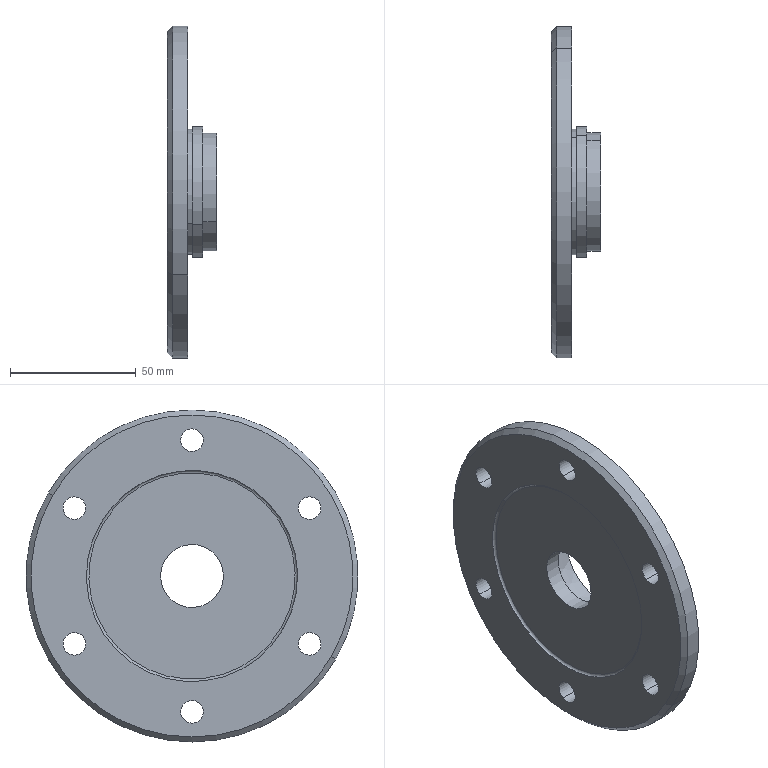Component | SolidWorks | HighSpeedAxisEndCoverA-1 | 1 solid | 37 faces | box 19.5 x 132 x 132 mm | volume 105490 mm3 | cylinder 22 | plane 7 | torus 4 | cone 4 | commonest cylinder face diameters 9 x12 25 x2 47 x2 50 x2 132 x2 52 x2
STEP:
#1=COLOUR_RGB('',0.7922,0.8196,0.9333);
#2=FILL_AREA_STYLE_COLOUR('',#1);
#3=FILL_AREA_STYLE('',(#2));
#4=SURFACE_STYLE_FILL_AREA(#3);
#5=SURFACE_SIDE_STYLE('',(#4));
#6=SURFACE_STYLE_USAGE(.BOTH.,#5);
#7=PRESENTATION_STYLE_ASSIGNMENT((#6));
#8=CARTESIAN_POINT('',(-19.213,0.6247,0.3607));
#9=VERTEX_POINT('',#8);
#10=CARTESIAN_POINT('',(-19.213,-0.6247,-0.3607));
#11=VERTEX_POINT('',#10);
#12=CARTESIAN_POINT('',(-19.213,0.,0.));
#13=DIRECTION('',(-1.,-0.,-0.));
#14=DIRECTION('',(0.,0.866,0.5));
#15=AXIS2_PLACEMENT_3D('',#12,#13,#14);
#16=CIRCLE('',#15,0.7213);
#17=EDGE_CURVE('',#9,#11,#16,.T.);
#18=ORIENTED_EDGE('',*,*,#17,.F.);
#19=CARTESIAN_POINT('',(-19.311,0.5239,0.3025));
#20=VERTEX_POINT('',#19);
#21=CARTESIAN_POINT('',(-19.193,0.5239,0.3025));
#22=DIRECTION('',(-0.,-0.5,0.866));
#23=DIRECTION('',(0.,-0.866,-0.5));
#24=AXIS2_PLACEMENT_3D('',#21,#22,#23);
#25=CIRCLE('',#24,0.1181);
#26=EDGE_CURVE('',#9,#20,#25,.T.);
#27=ORIENTED_EDGE('',*,*,#26,.T.);
#28=CARTESIAN_POINT('',(-19.311,-0.5239,-0.3025));
#29=VERTEX_POINT('',#28);
#30=CARTESIAN_POINT('',(-19.311,0.,0.));
#31=DIRECTION('',(1.,0.,0.));
#32=DIRECTION('',(0.,-0.866,-0.5));
#33=AXIS2_PLACEMENT_3D('',#30,#31,#32);
#34=CIRCLE('',#33,0.605);
#35=EDGE_CURVE('',#29,#20,#34,.T.);
#36=ORIENTED_EDGE('',*,*,#35,.F.);
#37=CARTESIAN_POINT('',(-19.193,-0.5239,-0.3025));
#38=DIRECTION('',(0.,0.5,-0.866));
#39=DIRECTION('',(0.,0.866,0.5));
#40=AXIS2_PLACEMENT_3D('',#37,#38,#39);
#41=CIRCLE('',#40,0.1181);
#42=EDGE_CURVE('',#11,#29,#41,.T.);
#43=ORIENTED_EDGE('',*,*,#42,.F.);
#44=EDGE_LOOP('',(#18,#27,#36,#43));
#45=FACE_OUTER_BOUND('',#44,.T.);
#46=CARTESIAN_POINT('',(-19.193,0.,0.));
#47=DIRECTION('',(-1.,-0.,-0.));
#48=DIRECTION('',(0.,-0.866,-0.5));
#49=AXIS2_PLACEMENT_3D('',#46,#47,#48);
#50=TOROIDAL_SURFACE('',#49,0.605,0.1181);
#51=ADVANCED_FACE('',(#45),#50,.F.);
#52=CARTESIAN_POINT('',(-19.606,-2.182,-1.26));
#53=VERTEX_POINT('',#52);
#54=CARTESIAN_POINT('',(-19.606,2.182,1.26));
#55=VERTEX_POINT('',#54);
#56=CARTESIAN_POINT('',(-19.606,0.,0.));
#57=DIRECTION('',(-1.,0.,0.));
#58=DIRECTION('',(0.,-0.866,-0.5));
#59=AXIS2_PLACEMENT_3D('',#56,#57,#58);
#60=CIRCLE('',#59,2.52);
#61=EDGE_CURVE('',#53,#55,#60,.T.);
#62=ORIENTED_EDGE('',*,*,#61,.F.);
#63=CARTESIAN_POINT('',(-19.528,-2.25,-1.299));
#64=VERTEX_POINT('',#63);
#65=CARTESIAN_POINT('',(-19.606,-2.182,-1.26));
#66=DIRECTION('',(0.7071,-0.6124,-0.3536));
#67=VECTOR('',#66,39.37);
#68=LINE('',#65,#67);
#69=EDGE_CURVE('',#53,#64,#68,.T.);
#70=ORIENTED_EDGE('',*,*,#69,.T.);
#71=CARTESIAN_POINT('',(-19.528,2.25,1.299));
#72=VERTEX_POINT('',#71);
#73=CARTESIAN_POINT('',(-19.528,0.,0.));
#74=DIRECTION('',(1.,-0.,-0.));
#75=DIRECTION('',(0.,-0.866,-0.5));
#76=AXIS2_PLACEMENT_3D('',#73,#74,#75);
#77=CIRCLE('',#76,2.598);
#78=EDGE_CURVE('',#72,#64,#77,.T.);
#79=ORIENTED_EDGE('',*,*,#78,.F.);
#80=CARTESIAN_POINT('',(-19.606,2.182,1.26));
#81=DIRECTION('',(0.7071,0.6124,0.3536));
#82=VECTOR('',#81,39.37);
#83=LINE('',#80,#82);
#84=EDGE_CURVE('',#55,#72,#83,.T.);
#85=ORIENTED_EDGE('',*,*,#84,.F.);
#86=EDGE_LOOP('',(#62,#70,#79,#85));
#87=FACE_OUTER_BOUND('',#86,.T.);
#88=CARTESIAN_POINT('',(-19.606,0.,0.));
#89=DIRECTION('',(1.,-0.,-0.));
#90=DIRECTION('',(0.,0.866,0.5));
#91=AXIS2_PLACEMENT_3D('',#88,#89,#90);
#92=CONICAL_SURFACE('',#91,2.52,0.7854);
#93=ADVANCED_FACE('',(#87),#92,.T.);
#94=CARTESIAN_POINT('',(-19.291,1.753,-0.9096));
#95=VERTEX_POINT('',#94);
#96=CARTESIAN_POINT('',(-19.291,1.93,-1.216));
#97=VERTEX_POINT('',#96);
#98=CARTESIAN_POINT('',(-19.291,1.841,-1.063));
#99=DIRECTION('',(1.,-0.,-0.));
#100=DIRECTION('',(0.,0.866,0.5));
#101=AXIS2_PLACEMENT_3D('',#98,#99,#100);
#102=CIRCLE('',#101,0.1772);
#103=EDGE_CURVE('',#95,#97,#102,.T.);
#104=ORIENTED_EDGE('',*,*,#103,.T.);
#105=CARTESIAN_POINT('',(-19.606,1.93,-1.216));
#106=VERTEX_POINT('',#105);
#107=CARTESIAN_POINT('',(-19.606,1.93,-1.216));
#108=DIRECTION('',(-1.,0.,-0.));
#109=VECTOR('',#108,39.37);
#110=LINE('',#107,#109);
#111=EDGE_CURVE('',#97,#106,#110,.T.);
#112=ORIENTED_EDGE('',*,*,#111,.T.);
#113=CARTESIAN_POINT('',(-19.606,1.753,-0.9096));
#114=VERTEX_POINT('',#113);
#115=CARTESIAN_POINT('',(-19.606,1.841,-1.063));
#116=DIRECTION('',(-1.,0.,-0.));
#117=DIRECTION('',(0.,-0.5,0.866));
#118=AXIS2_PLACEMENT_3D('',#115,#116,#117);
#119=CIRCLE('',#118,0.1772);
#120=EDGE_CURVE('',#106,#114,#119,.T.);
#121=ORIENTED_EDGE('',*,*,#120,.T.);
#122=CARTESIAN_POINT('',(-19.606,1.753,-0.9096));
#123=DIRECTION('',(-1.,0.,-0.));
#124=VECTOR('',#123,39.37);
#125=LINE('',#122,#124);
#126=EDGE_CURVE('',#95,#114,#125,.T.);
#127=ORIENTED_EDGE('',*,*,#126,.F.);
#128=EDGE_LOOP('',(#104,#112,#121,#127));
#129=FACE_OUTER_BOUND('',#128,.T.);
#130=CARTESIAN_POINT('',(-19.606,1.841,-1.063));
#131=DIRECTION('',(-1.,0.,-0.));
#132=DIRECTION('',(0.,-0.5,0.866));
#133=AXIS2_PLACEMENT_3D('',#130,#131,#132);
#134=CYLINDRICAL_SURFACE('',#133,0.1772);
#135=ADVANCED_FACE('',(#129),#134,.F.);
#136=CARTESIAN_POINT('',(-19.291,-0.08858,-1.973));
#137=VERTEX_POINT('',#136);
#138=CARTESIAN_POINT('',(-19.291,0.08858,-2.279));
#139=VERTEX_POINT('',#138);
#140=CARTESIAN_POINT('',(-19.291,-0.,-2.126));
#141=DIRECTION('',(1.,-0.,-0.));
#142=DIRECTION('',(0.,0.866,0.5));
#143=AXIS2_PLACEMENT_3D('',#140,#141,#142);
#144=CIRCLE('',#143,0.1772);
#145=EDGE_CURVE('',#137,#139,#144,.T.);
#146=ORIENTED_EDGE('',*,*,#145,.T.);
#147=CARTESIAN_POINT('',(-19.606,0.08858,-2.279));
#148=VERTEX_POINT('',#147);
#149=CARTESIAN_POINT('',(-19.606,0.08858,-2.279));
#150=DIRECTION('',(-1.,0.,-0.));
#151=VECTOR('',#150,39.37);
#152=LINE('',#149,#151);
#153=EDGE_CURVE('',#139,#148,#152,.T.);
#154=ORIENTED_EDGE('',*,*,#153,.T.);
#155=CARTESIAN_POINT('',(-19.606,-0.08858,-1.973));
#156=VERTEX_POINT('',#155);
#157=CARTESIAN_POINT('',(-19.606,-0.,-2.126));
#158=DIRECTION('',(-1.,0.,-0.));
#159=DIRECTION('',(0.,-0.5,0.866));
#160=AXIS2_PLACEMENT_3D('',#157,#158,#159);
#161=CIRCLE('',#160,0.1772);
#162=EDGE_CURVE('',#148,#156,#161,.T.);
#163=ORIENTED_EDGE('',*,*,#162,.T.);
#164=CARTESIAN_POINT('',(-19.606,-0.08858,-1.973));
#165=DIRECTION('',(-1.,0.,-0.));
#166=VECTOR('',#165,39.37);
#167=LINE('',#164,#166);
#168=EDGE_CURVE('',#137,#156,#167,.T.);
#169=ORIENTED_EDGE('',*,*,#168,.F.);
#170=EDGE_LOOP('',(#146,#154,#163,#169));
#171=FACE_OUTER_BOUND('',#170,.T.);
#172=CARTESIAN_POINT('',(-19.606,-0.,-2.126));
#173=DIRECTION('',(-1.,0.,-0.));
#174=DIRECTION('',(0.,-0.5,0.866));
#175=AXIS2_PLACEMENT_3D('',#172,#173,#174);
#176=CYLINDRICAL_SURFACE('',#175,0.1772);
#177=ADVANCED_FACE('',(#171),#176,.F.);
#178=CARTESIAN_POINT('',(-19.291,-1.93,-0.9096));
#179=VERTEX_POINT('',#178);
#180=CARTESIAN_POINT('',(-19.291,-1.753,-1.216));
#181=VERTEX_POINT('',#180);
#182=CARTESIAN_POINT('',(-19.291,-1.841,-1.063));
#183=DIRECTION('',(1.,-0.,-0.));
#184=DIRECTION('',(0.,0.866,0.5));
#185=AXIS2_PLACEMENT_3D('',#182,#183,#184);
#186=CIRCLE('',#185,0.1772);
#187=EDGE_CURVE('',#179,#181,#186,.T.);
#188=ORIENTED_EDGE('',*,*,#187,.T.);
#189=CARTESIAN_POINT('',(-19.606,-1.753,-1.216));
#190=VERTEX_POINT('',#189);
#191=CARTESIAN_POINT('',(-19.606,-1.753,-1.216));
#192=DIRECTION('',(-1.,0.,-0.));
#193=VECTOR('',#192,39.37);
#194=LINE('',#191,#193);
#195=EDGE_CURVE('',#181,#190,#194,.T.);
#196=ORIENTED_EDGE('',*,*,#195,.T.);
#197=CARTESIAN_POINT('',(-19.606,-1.93,-0.9096));
#198=VERTEX_POINT('',#197);
#199=CARTESIAN_POINT('',(-19.606,-1.841,-1.063));
#200=DIRECTION('',(-1.,0.,-0.));
#201=DIRECTION('',(0.,-0.5,0.866));
#202=AXIS2_PLACEMENT_3D('',#199,#200,#201);
#203=CIRCLE('',#202,0.1772);
#204=EDGE_CURVE('',#190,#198,#203,.T.);
#205=ORIENTED_EDGE('',*,*,#204,.T.);
#206=CARTESIAN_POINT('',(-19.606,-1.93,-0.9096));
#207=DIRECTION('',(-1.,0.,-0.));
#208=VECTOR('',#207,39.37);
#209=LINE('',#206,#208);
#210=EDGE_CURVE('',#179,#198,#209,.T.);
#211=ORIENTED_EDGE('',*,*,#210,.F.);
#212=EDGE_LOOP('',(#188,#196,#205,#211));
#213=FACE_OUTER_BOUND('',#212,.T.);
#214=CARTESIAN_POINT('',(-19.606,-1.841,-1.063));
#215=DIRECTION('',(-1.,0.,-0.));
#216=DIRECTION('',(0.,-0.5,0.866));
#217=AXIS2_PLACEMENT_3D('',#214,#215,#216);
#218=CYLINDRICAL_SURFACE('',#217,0.1772);
#219=ADVANCED_FACE('',(#213),#218,.F.);
#220=CARTESIAN_POINT('',(-19.291,-1.93,1.216));
#221=VERTEX_POINT('',#220);
#222=CARTESIAN_POINT('',(-19.291,-1.753,0.9096));
#223=VERTEX_POINT('',#222);
#224=CARTESIAN_POINT('',(-19.291,-1.841,1.063));
#225=DIRECTION('',(1.,-0.,-0.));
#226=DIRECTION('',(0.,0.866,0.5));
#227=AXIS2_PLACEMENT_3D('',#224,#225,#226);
#228=CIRCLE('',#227,0.1772);
#229=EDGE_CURVE('',#221,#223,#228,.T.);
#230=ORIENTED_EDGE('',*,*,#229,.T.);
#231=CARTESIAN_POINT('',(-19.606,-1.753,0.9096));
#232=VERTEX_POINT('',#231);
#233=CARTESIAN_POINT('',(-19.606,-1.753,0.9096));
#234=DIRECTION('',(-1.,-0.,-0.));
#235=VECTOR('',#234,39.37);
#236=LINE('',#233,#235);
#237=EDGE_CURVE('',#223,#232,#236,.T.);
#238=ORIENTED_EDGE('',*,*,#237,.T.);
#239=CARTESIAN_POINT('',(-19.606,-1.93,1.216));
#240=VERTEX_POINT('',#239);
#241=CARTESIAN_POINT('',(-19.606,-1.841,1.063));
#242=DIRECTION('',(-1.,-0.,-0.));
#243=DIRECTION('',(0.,-0.5,0.866));
#244=AXIS2_PLACEMENT_3D('',#241,#242,#243);
#245=CIRCLE('',#244,0.1772);
#246=EDGE_CURVE('',#232,#240,#245,.T.);
#247=ORIENTED_EDGE('',*,*,#246,.T.);
#248=CARTESIAN_POINT('',(-19.606,-1.93,1.216));
#249=DIRECTION('',(-1.,-0.,-0.));
#250=VECTOR('',#249,39.37);
#251=LINE('',#248,#250);
#252=EDGE_CURVE('',#221,#240,#251,.T.);
#253=ORIENTED_EDGE('',*,*,#252,.F.);
#254=EDGE_LOOP('',(#230,#238,#247,#253));
#255=FACE_OUTER_BOUND('',#254,.T.);
#256=CARTESIAN_POINT('',(-19.606,-1.841,1.063));
#257=DIRECTION('',(-1.,-0.,-0.));
#258=DIRECTION('',(0.,-0.5,0.866));
#259=AXIS2_PLACEMENT_3D('',#256,#257,#258);
#260=CYLINDRICAL_SURFACE('',#259,0.1772);
#261=ADVANCED_FACE('',(#255),#260,.F.);
#262=CARTESIAN_POINT('',(-19.291,-0.08858,2.279));
#263=VERTEX_POINT('',#262);
#264=CARTESIAN_POINT('',(-19.291,0.08858,1.973));
#265=VERTEX_POINT('',#264);
#266=CARTESIAN_POINT('',(-19.291,0.,2.126));
#267=DIRECTION('',(1.,-0.,-0.));
#268=DIRECTION('',(0.,0.866,0.5));
#269=AXIS2_PLACEMENT_3D('',#266,#267,#268);
#270=CIRCLE('',#269,0.1772);
#271=EDGE_CURVE('',#263,#265,#270,.T.);
#272=ORIENTED_EDGE('',*,*,#271,.T.);
#273=CARTESIAN_POINT('',(-19.606,0.08858,1.973));
#274=VERTEX_POINT('',#273);
#275=CARTESIAN_POINT('',(-19.606,0.08858,1.973));
#276=DIRECTION('',(-1.,-0.,-0.));
#277=VECTOR('',#276,39.37);
#278=LINE('',#275,#277);
#279=EDGE_CURVE('',#265,#274,#278,.T.);
#280=ORIENTED_EDGE('',*,*,#279,.T.);
#281=CARTESIAN_POINT('',(-19.606,-0.08858,2.279));
#282=VERTEX_POINT('',#281);
#283=CARTESIAN_POINT('',(-19.606,0.,2.126));
#284=DIRECTION('',(-1.,-0.,-0.));
#285=DIRECTION('',(0.,-0.5,0.866));
#286=AXIS2_PLACEMENT_3D('',#283,#284,#285);
#287=CIRCLE('',#286,0.1772);
#288=EDGE_CURVE('',#274,#282,#287,.T.);
#289=ORIENTED_EDGE('',*,*,#288,.T.);
#290=CARTESIAN_POINT('',(-19.606,-0.08858,2.279));
#291=DIRECTION('',(-1.,-0.,-0.));
#292=VECTOR('',#291,39.37);
#293=LINE('',#290,#292);
#294=EDGE_CURVE('',#263,#282,#293,.T.);
#295=ORIENTED_EDGE('',*,*,#294,.F.);
#296=EDGE_LOOP('',(#272,#280,#289,#295));
#297=FACE_OUTER_BOUND('',#296,.T.);
#298=CARTESIAN_POINT('',(-19.606,0.,2.126));
#299=DIRECTION('',(-1.,-0.,-0.));
#300=DIRECTION('',(0.,-0.5,0.866));
#301=AXIS2_PLACEMENT_3D('',#298,#299,#300);
#302=CYLINDRICAL_SURFACE('',#301,0.1772);
#303=ADVANCED_FACE('',(#297),#302,.F.);
#304=CARTESIAN_POINT('',(-19.291,1.753,1.216));
#305=VERTEX_POINT('',#304);
#306=CARTESIAN_POINT('',(-19.291,1.93,0.9096));
#307=VERTEX_POINT('',#306);
#308=CARTESIAN_POINT('',(-19.291,1.841,1.063));
#309=DIRECTION('',(1.,-0.,-0.));
#310=DIRECTION('',(0.,0.866,0.5));
#311=AXIS2_PLACEMENT_3D('',#308,#309,#310);
#312=CIRCLE('',#311,0.1772);
#313=EDGE_CURVE('',#305,#307,#312,.T.);
#314=ORIENTED_EDGE('',*,*,#313,.T.);
#315=CARTESIAN_POINT('',(-19.606,1.93,0.9096));
#316=VERTEX_POINT('',#315);
#317=CARTESIAN_POINT('',(-19.606,1.93,0.9096));
#318=DIRECTION('',(-1.,0.,-0.));
#319=VECTOR('',#318,39.37);
#320=LINE('',#317,#319);
#321=EDGE_CURVE('',#307,#316,#320,.T.);
#322=ORIENTED_EDGE('',*,*,#321,.T.);
#323=CARTESIAN_POINT('',(-19.606,1.753,1.216));
#324=VERTEX_POINT('',#323);
#325=CARTESIAN_POINT('',(-19.606,1.841,1.063));
#326=DIRECTION('',(-1.,0.,-0.));
#327=DIRECTION('',(0.,-0.5,0.866));
#328=AXIS2_PLACEMENT_3D('',#325,#326,#327);
#329=CIRCLE('',#328,0.1772);
#330=EDGE_CURVE('',#316,#324,#329,.T.);
#331=ORIENTED_EDGE('',*,*,#330,.T.);
#332=CARTESIAN_POINT('',(-19.606,1.753,1.216));
#333=DIRECTION('',(-1.,0.,-0.));
#334=VECTOR('',#333,39.37);
#335=LINE('',#332,#334);
#336=EDGE_CURVE('',#305,#324,#335,.T.);
#337=ORIENTED_EDGE('',*,*,#336,.F.);
#338=EDGE_LOOP('',(#314,#322,#331,#337));
#339=FACE_OUTER_BOUND('',#338,.T.);
#340=CARTESIAN_POINT('',(-19.606,1.841,1.063));
#341=DIRECTION('',(-1.,0.,-0.));
#342=DIRECTION('',(0.,-0.5,0.866));
#343=AXIS2_PLACEMENT_3D('',#340,#341,#342);
#344=CYLINDRICAL_SURFACE('',#343,0.1772);
#345=ADVANCED_FACE('',(#339),#344,.F.);
#346=CARTESIAN_POINT('',(-19.311,0.4262,0.2461));
#347=VERTEX_POINT('',#346);
#348=CARTESIAN_POINT('',(-19.311,-0.4262,-0.2461));
#349=VERTEX_POINT('',#348);
#350=CARTESIAN_POINT('',(-19.311,0.,0.));
#351=DIRECTION('',(-1.,-0.,-0.));
#352=DIRECTION('',(0.,-0.866,-0.5));
#353=AXIS2_PLACEMENT_3D('',#350,#351,#352);
#354=CIRCLE('',#353,0.4921);
#355=EDGE_CURVE('',#347,#349,#354,.T.);
#356=ORIENTED_EDGE('',*,*,#355,.F.);
#357=CARTESIAN_POINT('',(-19.567,0.4262,0.2461));
#358=VERTEX_POINT('',#357);
#359=CARTESIAN_POINT('',(-18.839,0.4262,0.2461));
#360=DIRECTION('',(-1.,-0.,-0.));
#361=VECTOR('',#360,39.37);
#362=LINE('',#359,#361);
#363=EDGE_CURVE('',#347,#358,#362,.T.);
#364=ORIENTED_EDGE('',*,*,#363,.T.);
#365=CARTESIAN_POINT('',(-19.567,-0.4262,-0.2461));
#366=VERTEX_POINT('',#365);
#367=CARTESIAN_POINT('',(-19.567,0.,0.));
#368=DIRECTION('',(-1.,-0.,-0.));
#369=DIRECTION('',(0.,-0.866,-0.5));
#370=AXIS2_PLACEMENT_3D('',#367,#368,#369);
#371=CIRCLE('',#370,0.4921);
#372=EDGE_CURVE('',#358,#366,#371,.T.);
#373=ORIENTED_EDGE('',*,*,#372,.T.);
#374=CARTESIAN_POINT('',(-18.839,-0.4262,-0.2461));
#375=DIRECTION('',(-1.,-0.,-0.));
#376=VECTOR('',#375,39.37);
#377=LINE('',#374,#376);
#378=EDGE_CURVE('',#349,#366,#377,.T.);
#379=ORIENTED_EDGE('',*,*,#378,.F.);
#380=EDGE_LOOP('',(#356,#364,#373,#379));
#381=FACE_OUTER_BOUND('',#380,.T.);
#382=CARTESIAN_POINT('',(-18.839,0.,0.));
#383=DIRECTION('',(-1.,-0.,-0.));
#384=DIRECTION('',(0.,-0.866,-0.5));
#385=AXIS2_PLACEMENT_3D('',#382,#383,#384);
#386=CYLINDRICAL_SURFACE('',#385,0.4921);
#387=ADVANCED_FACE('',(#381),#386,.F.);
#388=CARTESIAN_POINT('',(-19.567,1.398,0.8071));
#389=VERTEX_POINT('',#388);
#390=CARTESIAN_POINT('',(-19.567,-1.398,-0.8071));
#391=VERTEX_POINT('',#390);
#392=CARTESIAN_POINT('',(-19.567,0.,0.));
#393=DIRECTION('',(-1.,-0.,-0.));
#394=DIRECTION('',(0.,-0.866,-0.5));
#395=AXIS2_PLACEMENT_3D('',#392,#393,#394);
#396=CIRCLE('',#395,1.614);
#397=EDGE_CURVE('',#389,#391,#396,.T.);
#398=ORIENTED_EDGE('',*,*,#397,.F.);
#399=CARTESIAN_POINT('',(-19.606,1.432,0.8268));
#400=VERTEX_POINT('',#399);
#401=CARTESIAN_POINT('',(-19.606,1.398,0.8071));
#402=DIRECTION('',(-0.,-0.5,0.866));
#403=DIRECTION('',(0.,-0.866,-0.5));
#404=AXIS2_PLACEMENT_3D('',#401,#402,#403);
#405=CIRCLE('',#404,0.03937);
#406=EDGE_CURVE('',#389,#400,#405,.T.);
#407=ORIENTED_EDGE('',*,*,#406,.T.);
#408=CARTESIAN_POINT('',(-19.606,-1.432,-0.8268));
#409=VERTEX_POINT('',#408);
#410=CARTESIAN_POINT('',(-19.606,0.,0.));
#411=DIRECTION('',(-1.,-0.,-0.));
#412=DIRECTION('',(0.,-0.866,-0.5));
#413=AXIS2_PLACEMENT_3D('',#410,#411,#412);
#414=CIRCLE('',#413,1.654);
#415=EDGE_CURVE('',#400,#409,#414,.T.);
#416=ORIENTED_EDGE('',*,*,#415,.T.);
#417=CARTESIAN_POINT('',(-19.606,-1.398,-0.8071));
#418=DIRECTION('',(0.,0.5,-0.866));
#419=DIRECTION('',(0.,0.866,0.5));
#420=AXIS2_PLACEMENT_3D('',#417,#418,#419);
#421=CIRCLE('',#420,0.03937);
#422=EDGE_CURVE('',#391,#409,#421,.T.);
#423=ORIENTED_EDGE('',*,*,#422,.F.);
#424=EDGE_LOOP('',(#398,#407,#416,#423));
#425=FACE_OUTER_BOUND('',#424,.T.);
#426=CARTESIAN_POINT('',(-19.606,0.,0.));
#427=DIRECTION('',(-1.,-0.,-0.));
#428=DIRECTION('',(0.,-0.866,-0.5));
#429=AXIS2_PLACEMENT_3D('',#426,#427,#428);
#430=TOROIDAL_SURFACE('',#429,1.614,0.03937);
#431=ADVANCED_FACE('',(#425),#430,.F.);
#432=ORIENTED_EDGE('',*,*,#17,.T.);
#433=CARTESIAN_POINT('',(-18.839,-0.6819,-0.3937));
#434=VERTEX_POINT('',#433);
#435=CARTESIAN_POINT('',(-19.311,-0.6098,-0.352));
#436=DIRECTION('',(0.9848,-0.1504,-0.08682));
#437=VECTOR('',#436,39.37);
#438=LINE('',#435,#437);
#439=EDGE_CURVE('',#11,#434,#438,.T.);
#440=ORIENTED_EDGE('',*,*,#439,.T.);
#441=CARTESIAN_POINT('',(-18.839,0.6819,0.3937));
#442=VERTEX_POINT('',#441);
#443=CARTESIAN_POINT('',(-18.839,0.,0.));
#444=DIRECTION('',(-1.,-0.,-0.));
#445=DIRECTION('',(0.,-0.866,-0.5));
#446=AXIS2_PLACEMENT_3D('',#443,#444,#445);
#447=CIRCLE('',#446,0.7874);
#448=EDGE_CURVE('',#442,#434,#447,.T.);
#449=ORIENTED_EDGE('',*,*,#448,.F.);
#450=CARTESIAN_POINT('',(-19.311,0.6098,0.352));
#451=DIRECTION('',(0.9848,0.1504,0.08682));
#452=VECTOR('',#451,39.37);
#453=LINE('',#450,#452);
#454=EDGE_CURVE('',#9,#442,#453,.T.);
#455=ORIENTED_EDGE('',*,*,#454,.F.);
#456=EDGE_LOOP('',(#432,#440,#449,#455));
#457=FACE_OUTER_BOUND('',#456,.T.);
#458=CARTESIAN_POINT('',(-19.311,0.,0.));
#459=DIRECTION('',(1.,0.,0.));
#460=DIRECTION('',(0.,0.866,0.5));
#461=AXIS2_PLACEMENT_3D('',#458,#459,#460);
#462=CONICAL_SURFACE('',#461,0.7041,0.1745);
#463=ADVANCED_FACE('',(#457),#462,.F.);
#464=CARTESIAN_POINT('',(-18.839,0.8012,0.4626));
#465=VERTEX_POINT('',#464);
#466=CARTESIAN_POINT('',(-18.839,-0.8012,-0.4626));
#467=VERTEX_POINT('',#466);
#468=CARTESIAN_POINT('',(-18.839,0.,0.));
#469=DIRECTION('',(1.,-0.,-0.));
#470=DIRECTION('',(0.,0.866,0.5));
#471=AXIS2_PLACEMENT_3D('',#468,#469,#470);
#472=CIRCLE('',#471,0.9252);
#473=EDGE_CURVE('',#465,#467,#472,.T.);
#474=ORIENTED_EDGE('',*,*,#473,.F.);
#475=CARTESIAN_POINT('',(-19.055,0.8012,0.4626));
#476=VERTEX_POINT('',#475);
#477=CARTESIAN_POINT('',(-18.839,0.8012,0.4626));
#478=DIRECTION('',(-1.,0.,0.));
#479=VECTOR('',#478,39.37);
#480=LINE('',#477,#479);
#481=EDGE_CURVE('',#465,#476,#480,.T.);
#482=ORIENTED_EDGE('',*,*,#481,.T.);
#483=CARTESIAN_POINT('',(-19.055,-0.8012,-0.4626));
#484=VERTEX_POINT('',#483);
#485=CARTESIAN_POINT('',(-19.055,0.,0.));
#486=DIRECTION('',(1.,-0.,-0.));
#487=DIRECTION('',(0.,0.866,0.5));
#488=AXIS2_PLACEMENT_3D('',#485,#486,#487);
#489=CIRCLE('',#488,0.9252);
#490=EDGE_CURVE('',#476,#484,#489,.T.);
#491=ORIENTED_EDGE('',*,*,#490,.T.);
#492=CARTESIAN_POINT('',(-18.839,-0.8012,-0.4626));
#493=DIRECTION('',(-1.,0.,0.));
#494=VECTOR('',#493,39.37);
#495=LINE('',#492,#494);
#496=EDGE_CURVE('',#467,#484,#495,.T.);
#497=ORIENTED_EDGE('',*,*,#496,.F.);
#498=EDGE_LOOP('',(#474,#482,#491,#497));
#499=FACE_OUTER_BOUND('',#498,.T.);
#500=CARTESIAN_POINT('',(-18.839,0.,0.));
#501=DIRECTION('',(-1.,0.,0.));
#502=DIRECTION('',(0.,-0.866,-0.5));
#503=AXIS2_PLACEMENT_3D('',#500,#501,#502);
#504=CYLINDRICAL_SURFACE('',#503,0.9252);
#505=ADVANCED_FACE('',(#499),#504,.T.);
#506=CARTESIAN_POINT('',(-19.213,-0.8524,-0.4921));
#507=VERTEX_POINT('',#506);
#508=CARTESIAN_POINT('',(-19.213,0.8524,0.4921));
#509=VERTEX_POINT('',#508);
#510=CARTESIAN_POINT('',(-19.213,0.,0.));
#511=DIRECTION('',(-1.,0.,0.));
#512=DIRECTION('',(0.,-0.866,-0.5));
#513=AXIS2_PLACEMENT_3D('',#510,#511,#512);
#514=CIRCLE('',#513,0.9843);
#515=EDGE_CURVE('',#507,#509,#514,.T.);
#516=ORIENTED_EDGE('',*,*,#515,.T.);
#517=CARTESIAN_POINT('',(-19.291,0.8524,0.4921));
#518=VERTEX_POINT('',#517);
#519=CARTESIAN_POINT('',(-19.055,0.8524,0.4921));
#520=DIRECTION('',(-1.,0.,0.));
#521=VECTOR('',#520,39.37);
#522=LINE('',#519,#521);
#523=EDGE_CURVE('',#509,#518,#522,.T.);
#524=ORIENTED_EDGE('',*,*,#523,.T.);
#525=CARTESIAN_POINT('',(-19.291,-0.8524,-0.4921));
#526=VERTEX_POINT('',#525);
#527=CARTESIAN_POINT('',(-19.291,0.,0.));
#528=DIRECTION('',(-1.,0.,0.));
#529=DIRECTION('',(0.,-0.866,-0.5));
#530=AXIS2_PLACEMENT_3D('',#527,#528,#529);
#531=CIRCLE('',#530,0.9843);
#532=EDGE_CURVE('',#526,#518,#531,.T.);
#533=ORIENTED_EDGE('',*,*,#532,.F.);
#534=CARTESIAN_POINT('',(-19.055,-0.8524,-0.4921));
#535=DIRECTION('',(-1.,0.,0.));
#536=VECTOR('',#535,39.37);
#537=LINE('',#534,#536);
#538=EDGE_CURVE('',#507,#526,#537,.T.);
#539=ORIENTED_EDGE('',*,*,#538,.F.);
#540=EDGE_LOOP('',(#516,#524,#533,#539));
#541=FACE_OUTER_BOUND('',#540,.T.);
#542=CARTESIAN_POINT('',(-19.055,0.,0.));
#543=DIRECTION('',(-1.,0.,0.));
#544=DIRECTION('',(0.,-0.866,-0.5));
#545=AXIS2_PLACEMENT_3D('',#542,#543,#544);
#546=CYLINDRICAL_SURFACE('',#545,0.9843);
#547=ADVANCED_FACE('',(#541),#546,.T.);
#548=CARTESIAN_POINT('',(-19.291,-2.25,-1.299));
#549=VERTEX_POINT('',#548);
#550=CARTESIAN_POINT('',(-19.291,2.25,1.299));
#551=VERTEX_POINT('',#550);
#552=CARTESIAN_POINT('',(-19.291,0.,0.));
#553=DIRECTION('',(-1.,0.,0.));
#554=DIRECTION('',(0.,-0.866,-0.5));
#555=AXIS2_PLACEMENT_3D('',#552,#553,#554);
#556=CIRCLE('',#555,2.598);
#557=EDGE_CURVE('',#549,#551,#556,.T.);
#558=ORIENTED_EDGE('',*,*,#557,.T.);
#559=CARTESIAN_POINT('',(-19.055,2.25,1.299));
#560=DIRECTION('',(-1.,0.,0.));
#561=VECTOR('',#560,39.37);
#562=LINE('',#559,#561);
#563=EDGE_CURVE('',#551,#72,#562,.T.);
#564=ORIENTED_EDGE('',*,*,#563,.T.);
#565=ORIENTED_EDGE('',*,*,#78,.T.);
#566=CARTESIAN_POINT('',(-19.055,-2.25,-1.299));
#567=DIRECTION('',(-1.,0.,0.));
#568=VECTOR('',#567,39.37);
#569=LINE('',#566,#568);
#570=EDGE_CURVE('',#549,#64,#569,.T.);
#571=ORIENTED_EDGE('',*,*,#570,.F.);
#572=EDGE_LOOP('',(#558,#564,#565,#571));
#573=FACE_OUTER_BOUND('',#572,.T.);
#574=CARTESIAN_POINT('',(-19.055,0.,0.));
#575=DIRECTION('',(-1.,0.,0.));
#576=DIRECTION('',(0.,-0.866,-0.5));
#577=AXIS2_PLACEMENT_3D('',#574,#575,#576);
#578=CYLINDRICAL_SURFACE('',#577,2.598);
#579=ADVANCED_FACE('',(#573),#578,.T.);
#580=CARTESIAN_POINT('',(-19.055,-0.8865,-0.5118));
#581=VERTEX_POINT('',#580);
#582=CARTESIAN_POINT('',(-19.055,0.8865,0.5118));
#583=VERTEX_POINT('',#582);
#584=CARTESIAN_POINT('',(-19.055,0.,0.));
#585=DIRECTION('',(-1.,0.,0.));
#586=DIRECTION('',(0.,-0.866,-0.5));
#587=AXIS2_PLACEMENT_3D('',#584,#585,#586);
#588=CIRCLE('',#587,1.024);
#589=EDGE_CURVE('',#581,#583,#588,.T.);
#590=ORIENTED_EDGE('',*,*,#589,.T.);
#591=CARTESIAN_POINT('',(-19.213,0.8865,0.5118));
#592=VERTEX_POINT('',#591);
#593=CARTESIAN_POINT('',(-19.055,0.8865,0.5118));
#594=DIRECTION('',(-1.,0.,0.));
#595=VECTOR('',#594,39.37);
#596=LINE('',#593,#595);
#597=EDGE_CURVE('',#583,#592,#596,.T.);
#598=ORIENTED_EDGE('',*,*,#597,.T.);
#599=CARTESIAN_POINT('',(-19.213,-0.8865,-0.5118));
#600=VERTEX_POINT('',#599);
#601=CARTESIAN_POINT('',(-19.213,0.,0.));
#602=DIRECTION('',(-1.,0.,0.));
#603=DIRECTION('',(0.,-0.866,-0.5));
#604=AXIS2_PLACEMENT_3D('',#601,#602,#603);
#605=CIRCLE('',#604,1.024);
#606=EDGE_CURVE('',#600,#592,#605,.T.);
#607=ORIENTED_EDGE('',*,*,#606,.F.);
#608=CARTESIAN_POINT('',(-19.055,-0.8865,-0.5118));
#609=DIRECTION('',(-1.,0.,0.));
#610=VECTOR('',#609,39.37);
#611=LINE('',#608,#610);
#612=EDGE_CURVE('',#581,#600,#611,.T.);
#613=ORIENTED_EDGE('',*,*,#612,.F.);
#614=EDGE_LOOP('',(#590,#598,#607,#613));
#615=FACE_OUTER_BOUND('',#614,.T.);
#616=CARTESIAN_POINT('',(-19.055,0.,0.));
#617=DIRECTION('',(-1.,0.,0.));
#618=DIRECTION('',(0.,-0.866,-0.5));
#619=AXIS2_PLACEMENT_3D('',#616,#617,#618);
#620=CYLINDRICAL_SURFACE('',#619,1.024);
#621=ADVANCED_FACE('',(#615),#620,.T.);
#622=ORIENTED_EDGE('',*,*,#597,.F.);
#623=CARTESIAN_POINT('',(-19.055,0.,0.));
#624=DIRECTION('',(-1.,0.,0.));
#625=DIRECTION('',(0.,-0.866,-0.5));
#626=AXIS2_PLACEMENT_3D('',#623,#624,#625);
#627=CIRCLE('',#626,1.024);
#628=EDGE_CURVE('',#583,#581,#627,.T.);
#629=ORIENTED_EDGE('',*,*,#628,.T.);
#630=ORIENTED_EDGE('',*,*,#612,.T.);
#631=CARTESIAN_POINT('',(-19.213,0.,0.));
#632=DIRECTION('',(-1.,0.,0.));
#633=DIRECTION('',(0.,-0.866,-0.5));
#634=AXIS2_PLACEMENT_3D('',#631,#632,#633);
#635=CIRCLE('',#634,1.024);
#636=EDGE_CURVE('',#592,#600,#635,.T.);
#637=ORIENTED_EDGE('',*,*,#636,.F.);
#638=EDGE_LOOP('',(#622,#629,#630,#637));
#639=FACE_OUTER_BOUND('',#638,.T.);
#640=CARTESIAN_POINT('',(-19.055,0.,0.));
#641=DIRECTION('',(-1.,0.,0.));
#642=DIRECTION('',(0.,-0.866,-0.5));
#643=AXIS2_PLACEMENT_3D('',#640,#641,#642);
#644=CYLINDRICAL_SURFACE('',#643,1.024);
#645=ADVANCED_FACE('',(#639),#644,.T.);
#646=CARTESIAN_POINT('',(-19.055,0.,0.));
#647=DIRECTION('',(1.,-0.,-0.));
#648=DIRECTION('',(0.,0.866,0.5));
#649=AXIS2_PLACEMENT_3D('',#646,#647,#648);
#650=CIRCLE('',#649,0.9252);
#651=EDGE_CURVE('',#484,#476,#650,.T.);
#652=ORIENTED_EDGE('',*,*,#651,.F.);
#653=ORIENTED_EDGE('',*,*,#490,.F.);
#654=EDGE_LOOP('',(#652,#653));
#655=FACE_BOUND('',#654,.T.);
#656=ORIENTED_EDGE('',*,*,#589,.F.);
#657=ORIENTED_EDGE('',*,*,#628,.F.);
#658=EDGE_LOOP('',(#656,#657));
#659=FACE_OUTER_BOUND('',#658,.T.);
#660=CARTESIAN_POINT('',(-19.055,0.8865,0.5118));
#661=DIRECTION('',(1.,-0.,-0.));
#662=DIRECTION('',(0.,0.866,0.5));
#663=AXIS2_PLACEMENT_3D('',#660,#661,#662);
#664=PLANE('',#663);
#665=ADVANCED_FACE('',(#655,#659),#664,.T.);
#666=CARTESIAN_POINT('',(-19.606,0.,0.));
#667=DIRECTION('',(-1.,0.,0.));
#668=DIRECTION('',(0.,-0.866,-0.5));
#669=AXIS2_PLACEMENT_3D('',#666,#667,#668);
#670=CIRCLE('',#669,2.52);
#671=EDGE_CURVE('',#55,#53,#670,.T.);
#672=ORIENTED_EDGE('',*,*,#671,.T.);
#673=ORIENTED_EDGE('',*,*,#61,.T.);
#674=EDGE_LOOP('',(#672,#673));
#675=FACE_OUTER_BOUND('',#674,.T.);
#676=CARTESIAN_POINT('',(-19.606,1.841,-1.063));
#677=DIRECTION('',(-1.,0.,-0.));
#678=DIRECTION('',(0.,-0.5,0.866));
#679=AXIS2_PLACEMENT_3D('',#676,#677,#678);
#680=CIRCLE('',#679,0.1772);
#681=EDGE_CURVE('',#114,#106,#680,.T.);
#682=ORIENTED_EDGE('',*,*,#681,.F.);
#683=ORIENTED_EDGE('',*,*,#120,.F.);
#684=EDGE_LOOP('',(#682,#683));
#685=FACE_BOUND('',#684,.T.);
#686=CARTESIAN_POINT('',(-19.606,-0.,-2.126));
#687=DIRECTION('',(-1.,0.,-0.));
#688=DIRECTION('',(0.,-0.5,0.866));
#689=AXIS2_PLACEMENT_3D('',#686,#687,#688);
#690=CIRCLE('',#689,0.1772);
#691=EDGE_CURVE('',#156,#148,#690,.T.);
#692=ORIENTED_EDGE('',*,*,#691,.F.);
#693=ORIENTED_EDGE('',*,*,#162,.F.);
#694=EDGE_LOOP('',(#692,#693));
#695=FACE_BOUND('',#694,.T.);
#696=CARTESIAN_POINT('',(-19.606,-1.841,-1.063));
#697=DIRECTION('',(-1.,0.,-0.));
#698=DIRECTION('',(0.,-0.5,0.866));
#699=AXIS2_PLACEMENT_3D('',#696,#697,#698);
#700=CIRCLE('',#699,0.1772);
#701=EDGE_CURVE('',#198,#190,#700,.T.);
#702=ORIENTED_EDGE('',*,*,#701,.F.);
#703=ORIENTED_EDGE('',*,*,#204,.F.);
#704=EDGE_LOOP('',(#702,#703));
#705=FACE_BOUND('',#704,.T.);
#706=CARTESIAN_POINT('',(-19.606,-1.841,1.063));
#707=DIRECTION('',(-1.,-0.,-0.));
#708=DIRECTION('',(0.,-0.5,0.866));
#709=AXIS2_PLACEMENT_3D('',#706,#707,#708);
#710=CIRCLE('',#709,0.1772);
#711=EDGE_CURVE('',#240,#232,#710,.T.);
#712=ORIENTED_EDGE('',*,*,#711,.F.);
#713=ORIENTED_EDGE('',*,*,#246,.F.);
#714=EDGE_LOOP('',(#712,#713));
#715=FACE_BOUND('',#714,.T.);
#716=CARTESIAN_POINT('',(-19.606,0.,2.126));
#717=DIRECTION('',(-1.,-0.,-0.));
#718=DIRECTION('',(0.,-0.5,0.866));
#719=AXIS2_PLACEMENT_3D('',#716,#717,#718);
#720=CIRCLE('',#719,0.1772);
#721=EDGE_CURVE('',#282,#274,#720,.T.);
#722=ORIENTED_EDGE('',*,*,#721,.F.);
#723=ORIENTED_EDGE('',*,*,#288,.F.);
#724=EDGE_LOOP('',(#722,#723));
#725=FACE_BOUND('',#724,.T.);
#726=CARTESIAN_POINT('',(-19.606,1.841,1.063));
#727=DIRECTION('',(-1.,0.,-0.));
#728=DIRECTION('',(0.,-0.5,0.866));
#729=AXIS2_PLACEMENT_3D('',#726,#727,#728);
#730=CIRCLE('',#729,0.1772);
#731=EDGE_CURVE('',#324,#316,#730,.T.);
#732=ORIENTED_EDGE('',*,*,#731,.F.);
#733=ORIENTED_EDGE('',*,*,#330,.F.);
#734=EDGE_LOOP('',(#732,#733));
#735=FACE_BOUND('',#734,.T.);
#736=CARTESIAN_POINT('',(-19.606,0.,0.));
#737=DIRECTION('',(-1.,-0.,-0.));
#738=DIRECTION('',(0.,-0.866,-0.5));
#739=AXIS2_PLACEMENT_3D('',#736,#737,#738);
#740=CIRCLE('',#739,1.654);
#741=EDGE_CURVE('',#409,#400,#740,.T.);
#742=ORIENTED_EDGE('',*,*,#741,.F.);
#743=ORIENTED_EDGE('',*,*,#415,.F.);
#744=EDGE_LOOP('',(#742,#743));
#745=FACE_BOUND('',#744,.T.);
#746=CARTESIAN_POINT('',(-19.606,0.,0.));
#747=DIRECTION('',(-1.,0.,0.));
#748=DIRECTION('',(-0.,-0.866,-0.5));
#749=AXIS2_PLACEMENT_3D('',#746,#747,#748);
#750=PLANE('',#749);
#751=ADVANCED_FACE('',(#675,#685,#695,#705,#715,#725,#735,#745),#750,.T.);
#752=ORIENTED_EDGE('',*,*,#563,.F.);
#753=CARTESIAN_POINT('',(-19.291,0.,0.));
#754=DIRECTION('',(-1.,0.,0.));
#755=DIRECTION('',(0.,-0.866,-0.5));
#756=AXIS2_PLACEMENT_3D('',#753,#754,#755);
#757=CIRCLE('',#756,2.598);
#758=EDGE_CURVE('',#551,#549,#757,.T.);
#759=ORIENTED_EDGE('',*,*,#758,.T.);
#760=ORIENTED_EDGE('',*,*,#570,.T.);
#761=CARTESIAN_POINT('',(-19.528,0.,0.));
#762=DIRECTION('',(1.,-0.,-0.));
#763=DIRECTION('',(0.,-0.866,-0.5));
#764=AXIS2_PLACEMENT_3D('',#761,#762,#763);
#765=CIRCLE('',#764,2.598);
#766=EDGE_CURVE('',#64,#72,#765,.T.);
#767=ORIENTED_EDGE('',*,*,#766,.T.);
#768=EDGE_LOOP('',(#752,#759,#760,#767));
#769=FACE_OUTER_BOUND('',#768,.T.);
#770=CARTESIAN_POINT('',(-19.055,0.,0.));
#771=DIRECTION('',(-1.,0.,0.));
#772=DIRECTION('',(0.,-0.866,-0.5));
#773=AXIS2_PLACEMENT_3D('',#770,#771,#772);
#774=CYLINDRICAL_SURFACE('',#773,2.598);
#775=ADVANCED_FACE('',(#769),#774,.T.);
#776=ORIENTED_EDGE('',*,*,#103,.F.);
#777=CARTESIAN_POINT('',(-19.291,1.841,-1.063));
#778=DIRECTION('',(1.,-0.,-0.));
#779=DIRECTION('',(0.,0.866,0.5));
#780=AXIS2_PLACEMENT_3D('',#777,#778,#779);
#781=CIRCLE('',#780,0.1772);
#782=EDGE_CURVE('',#97,#95,#781,.T.);
#783=ORIENTED_EDGE('',*,*,#782,.F.);
#784=EDGE_LOOP('',(#776,#783));
#785=FACE_BOUND('',#784,.T.);
#786=ORIENTED_EDGE('',*,*,#145,.F.);
#787=CARTESIAN_POINT('',(-19.291,-0.,-2.126));
#788=DIRECTION('',(1.,-0.,-0.));
#789=DIRECTION('',(0.,0.866,0.5));
#790=AXIS2_PLACEMENT_3D('',#787,#788,#789);
#791=CIRCLE('',#790,0.1772);
#792=EDGE_CURVE('',#139,#137,#791,.T.);
#793=ORIENTED_EDGE('',*,*,#792,.F.);
#794=EDGE_LOOP('',(#786,#793));
#795=FACE_BOUND('',#794,.T.);
#796=ORIENTED_EDGE('',*,*,#187,.F.);
#797=CARTESIAN_POINT('',(-19.291,-1.841,-1.063));
#798=DIRECTION('',(1.,-0.,-0.));
#799=DIRECTION('',(0.,0.866,0.5));
#800=AXIS2_PLACEMENT_3D('',#797,#798,#799);
#801=CIRCLE('',#800,0.1772);
#802=EDGE_CURVE('',#181,#179,#801,.T.);
#803=ORIENTED_EDGE('',*,*,#802,.F.);
#804=EDGE_LOOP('',(#796,#803));
#805=FACE_BOUND('',#804,.T.);
#806=ORIENTED_EDGE('',*,*,#229,.F.);
#807=CARTESIAN_POINT('',(-19.291,-1.841,1.063));
#808=DIRECTION('',(1.,-0.,-0.));
#809=DIRECTION('',(0.,0.866,0.5));
#810=AXIS2_PLACEMENT_3D('',#807,#808,#809);
#811=CIRCLE('',#810,0.1772);
#812=EDGE_CURVE('',#223,#221,#811,.T.);
#813=ORIENTED_EDGE('',*,*,#812,.F.);
#814=EDGE_LOOP('',(#806,#813));
#815=FACE_BOUND('',#814,.T.);
#816=ORIENTED_EDGE('',*,*,#271,.F.);
#817=CARTESIAN_POINT('',(-19.291,0.,2.126));
#818=DIRECTION('',(1.,-0.,-0.));
#819=DIRECTION('',(0.,0.866,0.5));
#820=AXIS2_PLACEMENT_3D('',#817,#818,#819);
#821=CIRCLE('',#820,0.1772);
#822=EDGE_CURVE('',#265,#263,#821,.T.);
#823=ORIENTED_EDGE('',*,*,#822,.F.);
#824=EDGE_LOOP('',(#816,#823));
#825=FACE_BOUND('',#824,.T.);
#826=ORIENTED_EDGE('',*,*,#313,.F.);
#827=CARTESIAN_POINT('',(-19.291,1.841,1.063));
#828=DIRECTION('',(1.,-0.,-0.));
#829=DIRECTION('',(0.,0.866,0.5));
#830=AXIS2_PLACEMENT_3D('',#827,#828,#829);
#831=CIRCLE('',#830,0.1772);
#832=EDGE_CURVE('',#307,#305,#831,.T.);
#833=ORIENTED_EDGE('',*,*,#832,.F.);
#834=EDGE_LOOP('',(#826,#833));
#835=FACE_BOUND('',#834,.T.);
#836=ORIENTED_EDGE('',*,*,#532,.T.);
#837=CARTESIAN_POINT('',(-19.291,0.,0.));
#838=DIRECTION('',(-1.,0.,0.));
#839=DIRECTION('',(0.,-0.866,-0.5));
#840=AXIS2_PLACEMENT_3D('',#837,#838,#839);
#841=CIRCLE('',#840,0.9843);
#842=EDGE_CURVE('',#518,#526,#841,.T.);
#843=ORIENTED_EDGE('',*,*,#842,.T.);
#844=EDGE_LOOP('',(#836,#843));
#845=FACE_BOUND('',#844,.T.);
#846=ORIENTED_EDGE('',*,*,#557,.F.);
#847=ORIENTED_EDGE('',*,*,#758,.F.);
#848=EDGE_LOOP('',(#846,#847));
#849=FACE_OUTER_BOUND('',#848,.T.);
#850=CARTESIAN_POINT('',(-19.291,2.25,1.299));
#851=DIRECTION('',(1.,-0.,-0.));
#852=DIRECTION('',(0.,0.866,0.5));
#853=AXIS2_PLACEMENT_3D('',#850,#851,#852);
#854=PLANE('',#853);
#855=ADVANCED_FACE('',(#785,#795,#805,#815,#825,#835,#845,#849),#854,.T.);
#856=ORIENTED_EDGE('',*,*,#523,.F.);
#857=CARTESIAN_POINT('',(-19.213,0.,0.));
#858=DIRECTION('',(-1.,0.,0.));
#859=DIRECTION('',(0.,-0.866,-0.5));
#860=AXIS2_PLACEMENT_3D('',#857,#858,#859);
#861=CIRCLE('',#860,0.9843);
#862=EDGE_CURVE('',#509,#507,#861,.T.);
#863=ORIENTED_EDGE('',*,*,#862,.T.);
#864=ORIENTED_EDGE('',*,*,#538,.T.);
#865=ORIENTED_EDGE('',*,*,#842,.F.);
#866=EDGE_LOOP('',(#856,#863,#864,#865));
#867=FACE_OUTER_BOUND('',#866,.T.);
#868=CARTESIAN_POINT('',(-19.055,0.,0.));
#869=DIRECTION('',(-1.,0.,0.));
#870=DIRECTION('',(0.,-0.866,-0.5));
#871=AXIS2_PLACEMENT_3D('',#868,#869,#870);
#872=CYLINDRICAL_SURFACE('',#871,0.9843);
#873=ADVANCED_FACE('',(#867),#872,.T.);
#874=ORIENTED_EDGE('',*,*,#606,.T.);
#875=ORIENTED_EDGE('',*,*,#636,.T.);
#876=EDGE_LOOP('',(#874,#875));
#877=FACE_OUTER_BOUND('',#876,.T.);
#878=ORIENTED_EDGE('',*,*,#515,.F.);
#879=ORIENTED_EDGE('',*,*,#862,.F.);
#880=EDGE_LOOP('',(#878,#879));
#881=FACE_BOUND('',#880,.T.);
#882=CARTESIAN_POINT('',(-19.213,0.8524,0.4921));
#883=DIRECTION('',(-1.,0.,0.));
#884=DIRECTION('',(-0.,-0.866,-0.5));
#885=AXIS2_PLACEMENT_3D('',#882,#883,#884);
#886=PLANE('',#885);
#887=ADVANCED_FACE('',(#877,#881),#886,.T.);
#888=ORIENTED_EDGE('',*,*,#481,.F.);
#889=CARTESIAN_POINT('',(-18.839,0.,0.));
#890=DIRECTION('',(1.,-0.,-0.));
#891=DIRECTION('',(0.,0.866,0.5));
#892=AXIS2_PLACEMENT_3D('',#889,#890,#891);
#893=CIRCLE('',#892,0.9252);
#894=EDGE_CURVE('',#467,#465,#893,.T.);
#895=ORIENTED_EDGE('',*,*,#894,.F.);
#896=ORIENTED_EDGE('',*,*,#496,.T.);
#897=ORIENTED_EDGE('',*,*,#651,.T.);
#898=EDGE_LOOP('',(#888,#895,#896,#897));
#899=FACE_OUTER_BOUND('',#898,.T.);
#900=CARTESIAN_POINT('',(-18.839,0.,0.));
#901=DIRECTION('',(-1.,0.,0.));
#902=DIRECTION('',(0.,-0.866,-0.5));
#903=AXIS2_PLACEMENT_3D('',#900,#901,#902);
#904=CYLINDRICAL_SURFACE('',#903,0.9252);
#905=ADVANCED_FACE('',(#899),#904,.T.);
#906=ORIENTED_EDGE('',*,*,#448,.T.);
#907=CARTESIAN_POINT('',(-18.839,0.,0.));
#908=DIRECTION('',(-1.,-0.,-0.));
#909=DIRECTION('',(0.,-0.866,-0.5));
#910=AXIS2_PLACEMENT_3D('',#907,#908,#909);
#911=CIRCLE('',#910,0.7874);
#912=EDGE_CURVE('',#434,#442,#911,.T.);
#913=ORIENTED_EDGE('',*,*,#912,.T.);
#914=EDGE_LOOP('',(#906,#913));
#915=FACE_BOUND('',#914,.T.);
#916=ORIENTED_EDGE('',*,*,#894,.T.);
#917=ORIENTED_EDGE('',*,*,#473,.T.);
#918=EDGE_LOOP('',(#916,#917));
#919=FACE_OUTER_BOUND('',#918,.T.);
#920=CARTESIAN_POINT('',(-18.839,0.,0.));
#921=DIRECTION('',(1.,-0.,-0.));
#922=DIRECTION('',(0.,0.866,0.5));
#923=AXIS2_PLACEMENT_3D('',#920,#921,#922);
#924=PLANE('',#923);
#925=ADVANCED_FACE('',(#915,#919),#924,.T.);
#926=ORIENTED_EDGE('',*,*,#439,.F.);
#927=CARTESIAN_POINT('',(-19.213,0.,0.));
#928=DIRECTION('',(-1.,-0.,-0.));
#929=DIRECTION('',(0.,0.866,0.5));
#930=AXIS2_PLACEMENT_3D('',#927,#928,#929);
#931=CIRCLE('',#930,0.7213);
#932=EDGE_CURVE('',#11,#9,#931,.T.);
#933=ORIENTED_EDGE('',*,*,#932,.T.);
#934=ORIENTED_EDGE('',*,*,#454,.T.);
#935=ORIENTED_EDGE('',*,*,#912,.F.);
#936=EDGE_LOOP('',(#926,#933,#934,#935));
#937=FACE_OUTER_BOUND('',#936,.T.);
#938=CARTESIAN_POINT('',(-19.311,0.,0.));
#939=DIRECTION('',(1.,0.,0.));
#940=DIRECTION('',(0.,0.866,0.5));
#941=AXIS2_PLACEMENT_3D('',#938,#939,#940);
#942=CONICAL_SURFACE('',#941,0.7041,0.1745);
#943=ADVANCED_FACE('',(#937),#942,.F.);
#944=ORIENTED_EDGE('',*,*,#406,.F.);
#945=CARTESIAN_POINT('',(-19.567,0.,0.));
#946=DIRECTION('',(-1.,-0.,-0.));
#947=DIRECTION('',(0.,-0.866,-0.5));
#948=AXIS2_PLACEMENT_3D('',#945,#946,#947);
#949=CIRCLE('',#948,1.614);
#950=EDGE_CURVE('',#391,#389,#949,.T.);
#951=ORIENTED_EDGE('',*,*,#950,.F.);
#952=ORIENTED_EDGE('',*,*,#422,.T.);
#953=ORIENTED_EDGE('',*,*,#741,.T.);
#954=EDGE_LOOP('',(#944,#951,#952,#953));
#955=FACE_OUTER_BOUND('',#954,.T.);
#956=CARTESIAN_POINT('',(-19.606,0.,0.));
#957=DIRECTION('',(-1.,-0.,-0.));
#958=DIRECTION('',(0.,-0.866,-0.5));
#959=AXIS2_PLACEMENT_3D('',#956,#957,#958);
#960=TOROIDAL_SURFACE('',#959,1.614,0.03937);
#961=ADVANCED_FACE('',(#955),#960,.F.);
#962=CARTESIAN_POINT('',(-19.567,0.,0.));
#963=DIRECTION('',(-1.,-0.,-0.));
#964=DIRECTION('',(0.,-0.866,-0.5));
#965=AXIS2_PLACEMENT_3D('',#962,#963,#964);
#966=CIRCLE('',#965,0.4921);
#967=EDGE_CURVE('',#366,#358,#966,.T.);
#968=ORIENTED_EDGE('',*,*,#967,.F.);
#969=ORIENTED_EDGE('',*,*,#372,.F.);
#970=EDGE_LOOP('',(#968,#969));
#971=FACE_BOUND('',#970,.T.);
#972=ORIENTED_EDGE('',*,*,#950,.T.);
#973=ORIENTED_EDGE('',*,*,#397,.T.);
#974=EDGE_LOOP('',(#972,#973));
#975=FACE_OUTER_BOUND('',#974,.T.);
#976=CARTESIAN_POINT('',(-19.567,1.398,0.8071));
#977=DIRECTION('',(1.,0.,0.));
#978=DIRECTION('',(-0.,0.866,0.5));
#979=AXIS2_PLACEMENT_3D('',#976,#977,#978);
#980=PLANE('',#979);
#981=ADVANCED_FACE('',(#971,#975),#980,.F.);
#982=ORIENTED_EDGE('',*,*,#363,.F.);
#983=CARTESIAN_POINT('',(-19.311,0.,0.));
#984=DIRECTION('',(-1.,-0.,-0.));
#985=DIRECTION('',(0.,-0.866,-0.5));
#986=AXIS2_PLACEMENT_3D('',#983,#984,#985);
#987=CIRCLE('',#986,0.4921);
#988=EDGE_CURVE('',#349,#347,#987,.T.);
#989=ORIENTED_EDGE('',*,*,#988,.F.);
#990=ORIENTED_EDGE('',*,*,#378,.T.);
#991=ORIENTED_EDGE('',*,*,#967,.T.);
#992=EDGE_LOOP('',(#982,#989,#990,#991));
#993=FACE_OUTER_BOUND('',#992,.T.);
#994=CARTESIAN_POINT('',(-18.839,0.,0.));
#995=DIRECTION('',(-1.,-0.,-0.));
#996=DIRECTION('',(0.,-0.866,-0.5));
#997=AXIS2_PLACEMENT_3D('',#994,#995,#996);
#998=CYLINDRICAL_SURFACE('',#997,0.4921);
#999=ADVANCED_FACE('',(#993),#998,.F.);
#1000=ORIENTED_EDGE('',*,*,#35,.T.);
#1001=CARTESIAN_POINT('',(-19.311,0.,0.));
#1002=DIRECTION('',(1.,0.,0.));
#1003=DIRECTION('',(0.,-0.866,-0.5));
#1004=AXIS2_PLACEMENT_3D('',#1001,#1002,#1003);
#1005=CIRCLE('',#1004,0.605);
#1006=EDGE_CURVE('',#20,#29,#1005,.T.);
#1007=ORIENTED_EDGE('',*,*,#1006,.T.);
#1008=EDGE_LOOP('',(#1000,#1007));
#1009=FACE_OUTER_BOUND('',#1008,.T.);
#1010=ORIENTED_EDGE('',*,*,#988,.T.);
#1011=ORIENTED_EDGE('',*,*,#355,.T.);
#1012=EDGE_LOOP('',(#1010,#1011));
#1013=FACE_BOUND('',#1012,.T.);
#1014=CARTESIAN_POINT('',(-19.311,0.4262,0.2461));
#1015=DIRECTION('',(-1.,-0.,-0.));
#1016=DIRECTION('',(0.,-0.866,-0.5));
#1017=AXIS2_PLACEMENT_3D('',#1014,#1015,#1016);
#1018=PLANE('',#1017);
#1019=ADVANCED_FACE('',(#1009,#1013),#1018,.F.);
#1020=ORIENTED_EDGE('',*,*,#321,.F.);
#1021=ORIENTED_EDGE('',*,*,#832,.T.);
#1022=ORIENTED_EDGE('',*,*,#336,.T.);
#1023=ORIENTED_EDGE('',*,*,#731,.T.);
#1024=EDGE_LOOP('',(#1020,#1021,#1022,#1023));
#1025=FACE_OUTER_BOUND('',#1024,.T.);
#1026=CARTESIAN_POINT('',(-19.606,1.841,1.063));
#1027=DIRECTION('',(-1.,0.,-0.));
#1028=DIRECTION('',(0.,-0.5,0.866));
#1029=AXIS2_PLACEMENT_3D('',#1026,#1027,#1028);
#1030=CYLINDRICAL_SURFACE('',#1029,0.1772);
#1031=ADVANCED_FACE('',(#1025),#1030,.F.);
#1032=ORIENTED_EDGE('',*,*,#279,.F.);
#1033=ORIENTED_EDGE('',*,*,#822,.T.);
#1034=ORIENTED_EDGE('',*,*,#294,.T.);
#1035=ORIENTED_EDGE('',*,*,#721,.T.);
#1036=EDGE_LOOP('',(#1032,#1033,#1034,#1035));
#1037=FACE_OUTER_BOUND('',#1036,.T.);
#1038=CARTESIAN_POINT('',(-19.606,0.,2.126));
#1039=DIRECTION('',(-1.,-0.,-0.));
#1040=DIRECTION('',(0.,-0.5,0.866));
#1041=AXIS2_PLACEMENT_3D('',#1038,#1039,#1040);
#1042=CYLINDRICAL_SURFACE('',#1041,0.1772);
#1043=ADVANCED_FACE('',(#1037),#1042,.F.);
#1044=ORIENTED_EDGE('',*,*,#237,.F.);
#1045=ORIENTED_EDGE('',*,*,#812,.T.);
#1046=ORIENTED_EDGE('',*,*,#252,.T.);
#1047=ORIENTED_EDGE('',*,*,#711,.T.);
#1048=EDGE_LOOP('',(#1044,#1045,#1046,#1047));
#1049=FACE_OUTER_BOUND('',#1048,.T.);
#1050=CARTESIAN_POINT('',(-19.606,-1.841,1.063));
#1051=DIRECTION('',(-1.,-0.,-0.));
#1052=DIRECTION('',(0.,-0.5,0.866));
#1053=AXIS2_PLACEMENT_3D('',#1050,#1051,#1052);
#1054=CYLINDRICAL_SURFACE('',#1053,0.1772);
#1055=ADVANCED_FACE('',(#1049),#1054,.F.);
#1056=ORIENTED_EDGE('',*,*,#195,.F.);
#1057=ORIENTED_EDGE('',*,*,#802,.T.);
#1058=ORIENTED_EDGE('',*,*,#210,.T.);
#1059=ORIENTED_EDGE('',*,*,#701,.T.);
#1060=EDGE_LOOP('',(#1056,#1057,#1058,#1059));
#1061=FACE_OUTER_BOUND('',#1060,.T.);
#1062=CARTESIAN_POINT('',(-19.606,-1.841,-1.063));
#1063=DIRECTION('',(-1.,0.,-0.));
#1064=DIRECTION('',(0.,-0.5,0.866));
#1065=AXIS2_PLACEMENT_3D('',#1062,#1063,#1064);
#1066=CYLINDRICAL_SURFACE('',#1065,0.1772);
#1067=ADVANCED_FACE('',(#1061),#1066,.F.);
#1068=ORIENTED_EDGE('',*,*,#153,.F.);
#1069=ORIENTED_EDGE('',*,*,#792,.T.);
#1070=ORIENTED_EDGE('',*,*,#168,.T.);
#1071=ORIENTED_EDGE('',*,*,#691,.T.);
#1072=EDGE_LOOP('',(#1068,#1069,#1070,#1071));
#1073=FACE_OUTER_BOUND('',#1072,.T.);
#1074=CARTESIAN_POINT('',(-19.606,-0.,-2.126));
#1075=DIRECTION('',(-1.,0.,-0.));
#1076=DIRECTION('',(0.,-0.5,0.866));
#1077=AXIS2_PLACEMENT_3D('',#1074,#1075,#1076);
#1078=CYLINDRICAL_SURFACE('',#1077,0.1772);
#1079=ADVANCED_FACE('',(#1073),#1078,.F.);
#1080=ORIENTED_EDGE('',*,*,#111,.F.);
#1081=ORIENTED_EDGE('',*,*,#782,.T.);
#1082=ORIENTED_EDGE('',*,*,#126,.T.);
#1083=ORIENTED_EDGE('',*,*,#681,.T.);
#1084=EDGE_LOOP('',(#1080,#1081,#1082,#1083));
#1085=FACE_OUTER_BOUND('',#1084,.T.);
#1086=CARTESIAN_POINT('',(-19.606,1.841,-1.063));
#1087=DIRECTION('',(-1.,0.,-0.));
#1088=DIRECTION('',(0.,-0.5,0.866));
#1089=AXIS2_PLACEMENT_3D('',#1086,#1087,#1088);
#1090=CYLINDRICAL_SURFACE('',#1089,0.1772);
#1091=ADVANCED_FACE('',(#1085),#1090,.F.);
#1092=ORIENTED_EDGE('',*,*,#69,.F.);
#1093=ORIENTED_EDGE('',*,*,#671,.F.);
#1094=ORIENTED_EDGE('',*,*,#84,.T.);
#1095=ORIENTED_EDGE('',*,*,#766,.F.);
#1096=EDGE_LOOP('',(#1092,#1093,#1094,#1095));
#1097=FACE_OUTER_BOUND('',#1096,.T.);
#1098=CARTESIAN_POINT('',(-19.606,0.,0.));
#1099=DIRECTION('',(1.,-0.,-0.));
#1100=DIRECTION('',(0.,0.866,0.5));
#1101=AXIS2_PLACEMENT_3D('',#1098,#1099,#1100);
#1102=CONICAL_SURFACE('',#1101,2.52,0.7854);
#1103=ADVANCED_FACE('',(#1097),#1102,.T.);
#1104=ORIENTED_EDGE('',*,*,#26,.F.);
#1105=ORIENTED_EDGE('',*,*,#932,.F.);
#1106=ORIENTED_EDGE('',*,*,#42,.T.);
#1107=ORIENTED_EDGE('',*,*,#1006,.F.);
#1108=EDGE_LOOP('',(#1104,#1105,#1106,#1107));
#1109=FACE_OUTER_BOUND('',#1108,.T.);
#1110=CARTESIAN_POINT('',(-19.193,0.,0.));
#1111=DIRECTION('',(-1.,-0.,-0.));
#1112=DIRECTION('',(0.,-0.866,-0.5));
#1113=AXIS2_PLACEMENT_3D('',#1110,#1111,#1112);
#1114=TOROIDAL_SURFACE('',#1113,0.605,0.1181);
#1115=ADVANCED_FACE('',(#1109),#1114,.F.);
#1116=CLOSED_SHELL('',(#51,#93,#135,#177,#219,#261,#303,#345,#387,#431,#463,#505,#547,#579,#621,#645,#665,#751,#775,#855,#873,#887,#905,#925,#943,#961,#981,#999,#1019,#1031,#1043,#1055,#1067,#1079,#1091,#1103,#1115));
#1117=MANIFOLD_SOLID_BREP('',#1116);
#1118=STYLED_ITEM('',(#7),#1117);
#1119=PRESENTATION_LAYER_ASSIGNMENT('','',(#1118));
#1120=(LENGTH_UNIT()NAMED_UNIT(*)SI_UNIT($,.METRE.));
#1121=LENGTH_MEASURE_WITH_UNIT(LENGTH_MEASURE(0.0254),#1120);
#1122=DIMENSIONAL_EXPONENTS(1.,0.,0.,0.,0.,0.,0.);
#1123=(CONVERSION_BASED_UNIT('',#1121)LENGTH_UNIT()NAMED_UNIT(#1122));
#1124=UNCERTAINTY_MEASURE_WITH_UNIT(LENGTH_MEASURE(0.00001),#1123,'','');
#1125=(NAMED_UNIT(*)PLANE_ANGLE_UNIT()SI_UNIT($,.RADIAN.));
#1126=(NAMED_UNIT(*)SI_UNIT($,.STERADIAN.)SOLID_ANGLE_UNIT());
#1127=(GEOMETRIC_REPRESENTATION_CONTEXT(3)GLOBAL_UNCERTAINTY_ASSIGNED_CONTEXT((#1124))GLOBAL_UNIT_ASSIGNED_CONTEXT((#1123,#1125,#1126))REPRESENTATION_CONTEXT('',''));
#1128=MECHANICAL_DESIGN_GEOMETRIC_PRESENTATION_REPRESENTATION('',(#1118),#1127);
#1129=CARTESIAN_POINT('',(0.,0.,0.));
#1130=DIRECTION('',(0.,0.,1.));
#1131=DIRECTION('',(1.,0.,0.));
#1132=AXIS2_PLACEMENT_3D('',#1129,#1130,#1131);
#1133=(LENGTH_UNIT()NAMED_UNIT(*)SI_UNIT($,.METRE.));
#1134=LENGTH_MEASURE_WITH_UNIT(LENGTH_MEASURE(0.0254),#1133);
#1135=DIMENSIONAL_EXPONENTS(1.,0.,0.,0.,0.,0.,0.);
#1136=(CONVERSION_BASED_UNIT('',#1134)LENGTH_UNIT()NAMED_UNIT(#1135));
#1137=UNCERTAINTY_MEASURE_WITH_UNIT(LENGTH_MEASURE(0.00001),#1136,'','');
#1138=(NAMED_UNIT(*)PLANE_ANGLE_UNIT()SI_UNIT($,.RADIAN.));
#1139=(NAMED_UNIT(*)SI_UNIT($,.STERADIAN.)SOLID_ANGLE_UNIT());
#1140=(GEOMETRIC_REPRESENTATION_CONTEXT(3)GLOBAL_UNCERTAINTY_ASSIGNED_CONTEXT((#1137))GLOBAL_UNIT_ASSIGNED_CONTEXT((#1136,#1138,#1139))REPRESENTATION_CONTEXT('',''));
#1141=ADVANCED_BREP_SHAPE_REPRESENTATION('',(#1117,#1132),#1140);